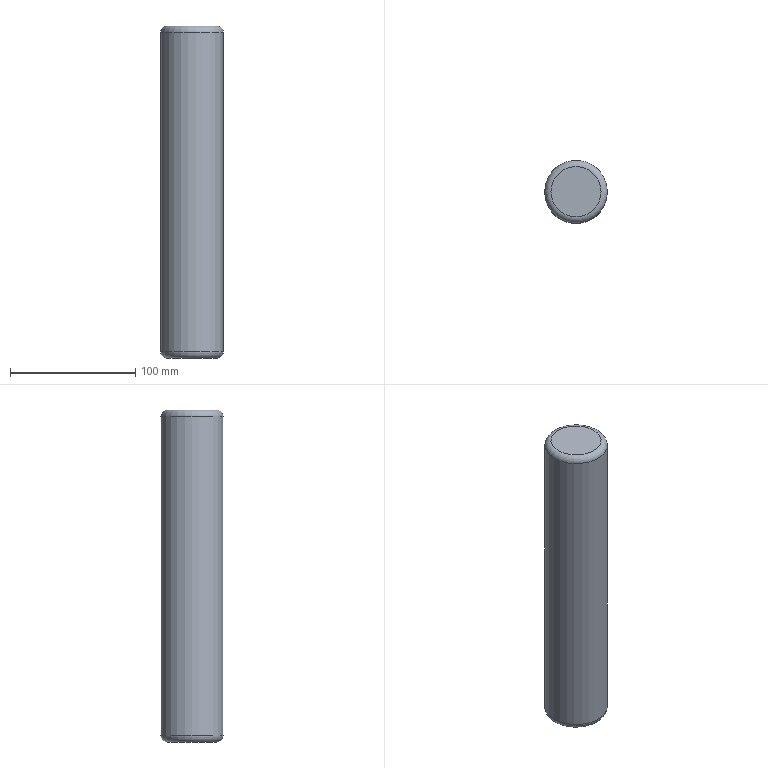Component | NX | OUTER_GUIDE_POST | 1 solid | 5 faces | box 50 x 50 x 265 mm | volume 518716 mm3 | plane 2 | torus 2 | cylinder 1 | commonest cylinder face diameters 50 x1
STEP:
#1=CARTESIAN_POINT('',(0.,0.,0.));
#2=DIRECTION('',(0.,0.,1.));
#3=DIRECTION('',(1.,0.,0.));
#4=AXIS2_PLACEMENT_3D('',#1,#2,#3);
#5=CARTESIAN_POINT('',(310.,290.,205.));
#6=VERTEX_POINT('',#5);
#7=CARTESIAN_POINT('',(290.,290.,205.));
#8=DIRECTION('',(0.,0.,1.));
#9=DIRECTION('',(1.,0.,0.));
#10=AXIS2_PLACEMENT_3D('',#7,#8,#9);
#11=CIRCLE('',#10,20.);
#12=CARTESIAN_POINT('',(290.,290.,205.));
#13=DIRECTION('',(0.,0.,1.));
#14=DIRECTION('',(1.,0.,0.));
#15=AXIS2_PLACEMENT_3D('',#12,#13,#14);
#16=PLANE('',#15);
#17=CARTESIAN_POINT('',(0.,0.));
#18=DIRECTION('',(1.,0.));
#19=AXIS2_PLACEMENT_2D('',#17,#18);
#20=CIRCLE('',#19,20.);
#21=(GEOMETRIC_REPRESENTATION_CONTEXT(2)PARAMETRIC_REPRESENTATION_CONTEXT()REPRESENTATION_CONTEXT('',''));
#22=DEFINITIONAL_REPRESENTATION('',(#20),#21);
#23=PCURVE('',#16,#22);
#24=CARTESIAN_POINT('',(290.,290.,200.));
#25=DIRECTION('',(0.,0.,1.));
#26=DIRECTION('',(1.,0.,0.));
#27=AXIS2_PLACEMENT_3D('',#24,#25,#26);
#28=TOROIDAL_SURFACE('',#27,20.,5.);
#29=CARTESIAN_POINT('',(0.,7.854));
#30=DIRECTION('',(1.,0.));
#31=VECTOR('',#30,1.);
#32=LINE('',#29,#31);
#33=(GEOMETRIC_REPRESENTATION_CONTEXT(2)PARAMETRIC_REPRESENTATION_CONTEXT()REPRESENTATION_CONTEXT('',''));
#34=DEFINITIONAL_REPRESENTATION('',(#32),#33);
#35=PCURVE('',#28,#34);
#36=SURFACE_CURVE('',#11,(#23,#35),.PCURVE_S1.);
#37=EDGE_CURVE('',#6,#6,#36,.T.);
#38=ORIENTED_EDGE('',*,*,#37,.T.);
#39=EDGE_LOOP('',(#38));
#40=FACE_BOUND('',#39,.T.);
#41=ADVANCED_FACE('',(#40),#16,.T.);
#42=CARTESIAN_POINT('',(270.,290.,-60.));
#43=VERTEX_POINT('',#42);
#44=CARTESIAN_POINT('',(290.,290.,-60.));
#45=DIRECTION('',(0.,0.,-1.));
#46=DIRECTION('',(-1.,0.,0.));
#47=AXIS2_PLACEMENT_3D('',#44,#45,#46);
#48=CIRCLE('',#47,20.);
#49=CARTESIAN_POINT('',(290.,290.,-60.));
#50=DIRECTION('',(0.,0.,-1.));
#51=DIRECTION('',(-1.,0.,0.));
#52=AXIS2_PLACEMENT_3D('',#49,#50,#51);
#53=PLANE('',#52);
#54=CARTESIAN_POINT('',(0.,0.));
#55=DIRECTION('',(1.,0.));
#56=AXIS2_PLACEMENT_2D('',#54,#55);
#57=CIRCLE('',#56,20.);
#58=(GEOMETRIC_REPRESENTATION_CONTEXT(2)PARAMETRIC_REPRESENTATION_CONTEXT()REPRESENTATION_CONTEXT('',''));
#59=DEFINITIONAL_REPRESENTATION('',(#57),#58);
#60=PCURVE('',#53,#59);
#61=CARTESIAN_POINT('',(290.,290.,-55.));
#62=DIRECTION('',(0.,0.,-1.));
#63=DIRECTION('',(-1.,0.,0.));
#64=AXIS2_PLACEMENT_3D('',#61,#62,#63);
#65=TOROIDAL_SURFACE('',#64,20.,5.);
#66=CARTESIAN_POINT('',(0.,7.854));
#67=DIRECTION('',(1.,0.));
#68=VECTOR('',#67,1.);
#69=LINE('',#66,#68);
#70=(GEOMETRIC_REPRESENTATION_CONTEXT(2)PARAMETRIC_REPRESENTATION_CONTEXT()REPRESENTATION_CONTEXT('',''));
#71=DEFINITIONAL_REPRESENTATION('',(#69),#70);
#72=PCURVE('',#65,#71);
#73=SURFACE_CURVE('',#48,(#60,#72),.PCURVE_S1.);
#74=EDGE_CURVE('',#43,#43,#73,.T.);
#75=ORIENTED_EDGE('',*,*,#74,.T.);
#76=EDGE_LOOP('',(#75));
#77=FACE_BOUND('',#76,.T.);
#78=ADVANCED_FACE('',(#77),#53,.T.);
#79=CARTESIAN_POINT('',(315.,290.,200.));
#80=VERTEX_POINT('',#79);
#81=CARTESIAN_POINT('',(290.,290.,200.));
#82=DIRECTION('',(0.,0.,-1.));
#83=DIRECTION('',(1.,0.,0.));
#84=AXIS2_PLACEMENT_3D('',#81,#82,#83);
#85=CIRCLE('',#84,25.);
#86=CARTESIAN_POINT('',(290.,290.,-60.));
#87=DIRECTION('',(0.,0.,1.));
#88=DIRECTION('',(1.,0.,0.));
#89=AXIS2_PLACEMENT_3D('',#86,#87,#88);
#90=CYLINDRICAL_SURFACE('',#89,25.);
#91=CARTESIAN_POINT('',(6.283,260.));
#92=DIRECTION('',(-1.,0.));
#93=VECTOR('',#92,1.);
#94=LINE('',#91,#93);
#95=(GEOMETRIC_REPRESENTATION_CONTEXT(2)PARAMETRIC_REPRESENTATION_CONTEXT()REPRESENTATION_CONTEXT('',''));
#96=DEFINITIONAL_REPRESENTATION('',(#94),#95);
#97=PCURVE('',#90,#96);
#98=CARTESIAN_POINT('',(6.283,6.283));
#99=DIRECTION('',(-1.,0.));
#100=VECTOR('',#99,1.);
#101=LINE('',#98,#100);
#102=(GEOMETRIC_REPRESENTATION_CONTEXT(2)PARAMETRIC_REPRESENTATION_CONTEXT()REPRESENTATION_CONTEXT('',''));
#103=DEFINITIONAL_REPRESENTATION('',(#101),#102);
#104=PCURVE('',#28,#103);
#105=SURFACE_CURVE('',#85,(#97,#104),.PCURVE_S1.);
#106=EDGE_CURVE('',#80,#80,#105,.T.);
#107=ORIENTED_EDGE('',*,*,#106,.T.);
#108=CARTESIAN_POINT('',(315.,290.,-55.));
#109=VERTEX_POINT('',#108);
#110=CARTESIAN_POINT('',(315.,290.,-55.));
#111=CARTESIAN_POINT('',(315.,290.,200.));
#112=B_SPLINE_CURVE_WITH_KNOTS('',1,(#110,#111),.UNSPECIFIED.,.F.,.F.,(2,2),(5.,260.),.PIECEWISE_BEZIER_KNOTS.);
#113=CARTESIAN_POINT('',(0.,0.));
#114=DIRECTION('',(0.,1.));
#115=VECTOR('',#114,1.);
#116=LINE('',#113,#115);
#117=(GEOMETRIC_REPRESENTATION_CONTEXT(2)PARAMETRIC_REPRESENTATION_CONTEXT()REPRESENTATION_CONTEXT('',''));
#118=DEFINITIONAL_REPRESENTATION('',(#116),#117);
#119=PCURVE('',#90,#118);
#120=CARTESIAN_POINT('',(6.283,0.));
#121=DIRECTION('',(0.,1.));
#122=VECTOR('',#121,1.);
#123=LINE('',#120,#122);
#124=(GEOMETRIC_REPRESENTATION_CONTEXT(2)PARAMETRIC_REPRESENTATION_CONTEXT()REPRESENTATION_CONTEXT('',''));
#125=DEFINITIONAL_REPRESENTATION('',(#123),#124);
#126=PCURVE('',#90,#125);
#127=SEAM_CURVE('',#112,(#119,#126),.PCURVE_S1.);
#128=EDGE_CURVE('',#109,#80,#127,.T.);
#129=ORIENTED_EDGE('',*,*,#128,.F.);
#130=CARTESIAN_POINT('',(265.,290.,-55.));
#131=VERTEX_POINT('',#130);
#132=CARTESIAN_POINT('',(290.,290.,-55.));
#133=DIRECTION('',(0.,0.,1.));
#134=DIRECTION('',(-1.,0.,0.));
#135=AXIS2_PLACEMENT_3D('',#132,#133,#134);
#136=CIRCLE('',#135,25.);
#137=CARTESIAN_POINT('',(-3.142,5.));
#138=DIRECTION('',(1.,0.));
#139=VECTOR('',#138,1.);
#140=LINE('',#137,#139);
#141=(GEOMETRIC_REPRESENTATION_CONTEXT(2)PARAMETRIC_REPRESENTATION_CONTEXT()REPRESENTATION_CONTEXT('',''));
#142=DEFINITIONAL_REPRESENTATION('',(#140),#141);
#143=PCURVE('',#90,#142);
#144=CARTESIAN_POINT('',(6.283,6.283));
#145=DIRECTION('',(-1.,0.));
#146=VECTOR('',#145,1.);
#147=LINE('',#144,#146);
#148=(GEOMETRIC_REPRESENTATION_CONTEXT(2)PARAMETRIC_REPRESENTATION_CONTEXT()REPRESENTATION_CONTEXT('',''));
#149=DEFINITIONAL_REPRESENTATION('',(#147),#148);
#150=PCURVE('',#65,#149);
#151=SURFACE_CURVE('',#136,(#143,#150),.PCURVE_S1.);
#152=EDGE_CURVE('',#109,#131,#151,.T.);
#153=ORIENTED_EDGE('',*,*,#152,.T.);
#154=CARTESIAN_POINT('',(290.,290.,-55.));
#155=DIRECTION('',(0.,0.,1.));
#156=DIRECTION('',(-1.,0.,0.));
#157=AXIS2_PLACEMENT_3D('',#154,#155,#156);
#158=CIRCLE('',#157,25.);
#159=CARTESIAN_POINT('',(3.142,5.));
#160=DIRECTION('',(1.,0.));
#161=VECTOR('',#160,1.);
#162=LINE('',#159,#161);
#163=(GEOMETRIC_REPRESENTATION_CONTEXT(2)PARAMETRIC_REPRESENTATION_CONTEXT()REPRESENTATION_CONTEXT('',''));
#164=DEFINITIONAL_REPRESENTATION('',(#162),#163);
#165=PCURVE('',#90,#164);
#166=CARTESIAN_POINT('',(6.283,6.283));
#167=DIRECTION('',(-1.,0.));
#168=VECTOR('',#167,1.);
#169=LINE('',#166,#168);
#170=(GEOMETRIC_REPRESENTATION_CONTEXT(2)PARAMETRIC_REPRESENTATION_CONTEXT()REPRESENTATION_CONTEXT('',''));
#171=DEFINITIONAL_REPRESENTATION('',(#169),#170);
#172=PCURVE('',#65,#171);
#173=SURFACE_CURVE('',#158,(#165,#172),.PCURVE_S1.);
#174=EDGE_CURVE('',#131,#109,#173,.T.);
#175=ORIENTED_EDGE('',*,*,#174,.T.);
#176=ORIENTED_EDGE('',*,*,#128,.T.);
#177=EDGE_LOOP('',(#107,#129,#153,#175,#176));
#178=FACE_BOUND('',#177,.T.);
#179=ADVANCED_FACE('',(#178),#90,.T.);
#180=ORIENTED_EDGE('',*,*,#37,.F.);
#181=CARTESIAN_POINT('',(315.,290.,200.));
#182=CARTESIAN_POINT('',(315.,290.,201.337));
#183=CARTESIAN_POINT('',(314.575,290.,202.639));
#184=CARTESIAN_POINT('',(313.76,290.,203.76));
#185=CARTESIAN_POINT('',(312.639,290.,204.575));
#186=CARTESIAN_POINT('',(311.337,290.,205.));
#187=CARTESIAN_POINT('',(310.,290.,205.));
#188=(BOUNDED_CURVE()B_SPLINE_CURVE(6,(#181,#182,#183,#184,#185,#186,#187),.UNSPECIFIED.,.F.,.F.)B_SPLINE_CURVE_WITH_KNOTS((7,7),(0.,1.571),.PIECEWISE_BEZIER_KNOTS.)CURVE()GEOMETRIC_REPRESENTATION_ITEM()RATIONAL_B_SPLINE_CURVE((1.031,1.01,0.9979,0.994,0.9979,1.01,1.031))REPRESENTATION_ITEM(''));
#189=CARTESIAN_POINT('',(0.,6.283));
#190=DIRECTION('',(0.,1.));
#191=VECTOR('',#190,1.);
#192=LINE('',#189,#191);
#193=(GEOMETRIC_REPRESENTATION_CONTEXT(2)PARAMETRIC_REPRESENTATION_CONTEXT()REPRESENTATION_CONTEXT('',''));
#194=DEFINITIONAL_REPRESENTATION('',(#192),#193);
#195=PCURVE('',#28,#194);
#196=CARTESIAN_POINT('',(6.283,6.283));
#197=DIRECTION('',(0.,1.));
#198=VECTOR('',#197,1.);
#199=LINE('',#196,#198);
#200=(GEOMETRIC_REPRESENTATION_CONTEXT(2)PARAMETRIC_REPRESENTATION_CONTEXT()REPRESENTATION_CONTEXT('',''));
#201=DEFINITIONAL_REPRESENTATION('',(#199),#200);
#202=PCURVE('',#28,#201);
#203=SEAM_CURVE('',#188,(#195,#202),.PCURVE_S1.);
#204=EDGE_CURVE('',#80,#6,#203,.T.);
#205=ORIENTED_EDGE('',*,*,#204,.F.);
#206=ORIENTED_EDGE('',*,*,#106,.F.);
#207=ORIENTED_EDGE('',*,*,#204,.T.);
#208=EDGE_LOOP('',(#180,#205,#206,#207));
#209=FACE_BOUND('',#208,.T.);
#210=ADVANCED_FACE('',(#209),#28,.T.);
#211=ORIENTED_EDGE('',*,*,#74,.F.);
#212=CARTESIAN_POINT('',(265.,290.,-55.));
#213=CARTESIAN_POINT('',(265.,290.,-56.337));
#214=CARTESIAN_POINT('',(265.425,290.,-57.639));
#215=CARTESIAN_POINT('',(266.24,290.,-58.76));
#216=CARTESIAN_POINT('',(267.361,290.,-59.575));
#217=CARTESIAN_POINT('',(268.663,290.,-60.));
#218=CARTESIAN_POINT('',(270.,290.,-60.));
#219=(BOUNDED_CURVE()B_SPLINE_CURVE(6,(#212,#213,#214,#215,#216,#217,#218),.UNSPECIFIED.,.F.,.F.)B_SPLINE_CURVE_WITH_KNOTS((7,7),(0.,1.571),.PIECEWISE_BEZIER_KNOTS.)CURVE()GEOMETRIC_REPRESENTATION_ITEM()RATIONAL_B_SPLINE_CURVE((1.031,1.01,0.9979,0.994,0.9979,1.01,1.031))REPRESENTATION_ITEM(''));
#220=CARTESIAN_POINT('',(0.,6.283));
#221=DIRECTION('',(0.,1.));
#222=VECTOR('',#221,1.);
#223=LINE('',#220,#222);
#224=(GEOMETRIC_REPRESENTATION_CONTEXT(2)PARAMETRIC_REPRESENTATION_CONTEXT()REPRESENTATION_CONTEXT('',''));
#225=DEFINITIONAL_REPRESENTATION('',(#223),#224);
#226=PCURVE('',#65,#225);
#227=CARTESIAN_POINT('',(6.283,6.283));
#228=DIRECTION('',(0.,1.));
#229=VECTOR('',#228,1.);
#230=LINE('',#227,#229);
#231=(GEOMETRIC_REPRESENTATION_CONTEXT(2)PARAMETRIC_REPRESENTATION_CONTEXT()REPRESENTATION_CONTEXT('',''));
#232=DEFINITIONAL_REPRESENTATION('',(#230),#231);
#233=PCURVE('',#65,#232);
#234=SEAM_CURVE('',#219,(#226,#233),.PCURVE_S1.);
#235=EDGE_CURVE('',#131,#43,#234,.T.);
#236=ORIENTED_EDGE('',*,*,#235,.F.);
#237=ORIENTED_EDGE('',*,*,#152,.F.);
#238=ORIENTED_EDGE('',*,*,#174,.F.);
#239=ORIENTED_EDGE('',*,*,#235,.T.);
#240=EDGE_LOOP('',(#211,#236,#237,#238,#239));
#241=FACE_BOUND('',#240,.T.);
#242=ADVANCED_FACE('',(#241),#65,.T.);
#243=CLOSED_SHELL('',(#41,#78,#179,#210,#242));
#244=MANIFOLD_SOLID_BREP('',#243);
#245=(LENGTH_UNIT()NAMED_UNIT(*)SI_UNIT(.MILLI.,.METRE.));
#246=UNCERTAINTY_MEASURE_WITH_UNIT(LENGTH_MEASURE(0.00001),#245,'','');
#247=(NAMED_UNIT(*)PLANE_ANGLE_UNIT()SI_UNIT($,.RADIAN.));
#248=(NAMED_UNIT(*)SI_UNIT($,.STERADIAN.)SOLID_ANGLE_UNIT());
#249=(GEOMETRIC_REPRESENTATION_CONTEXT(3)GLOBAL_UNCERTAINTY_ASSIGNED_CONTEXT((#246))GLOBAL_UNIT_ASSIGNED_CONTEXT((#245,#247,#248))REPRESENTATION_CONTEXT('',''));
#250=ADVANCED_BREP_SHAPE_REPRESENTATION('',(#4,#244),#249);